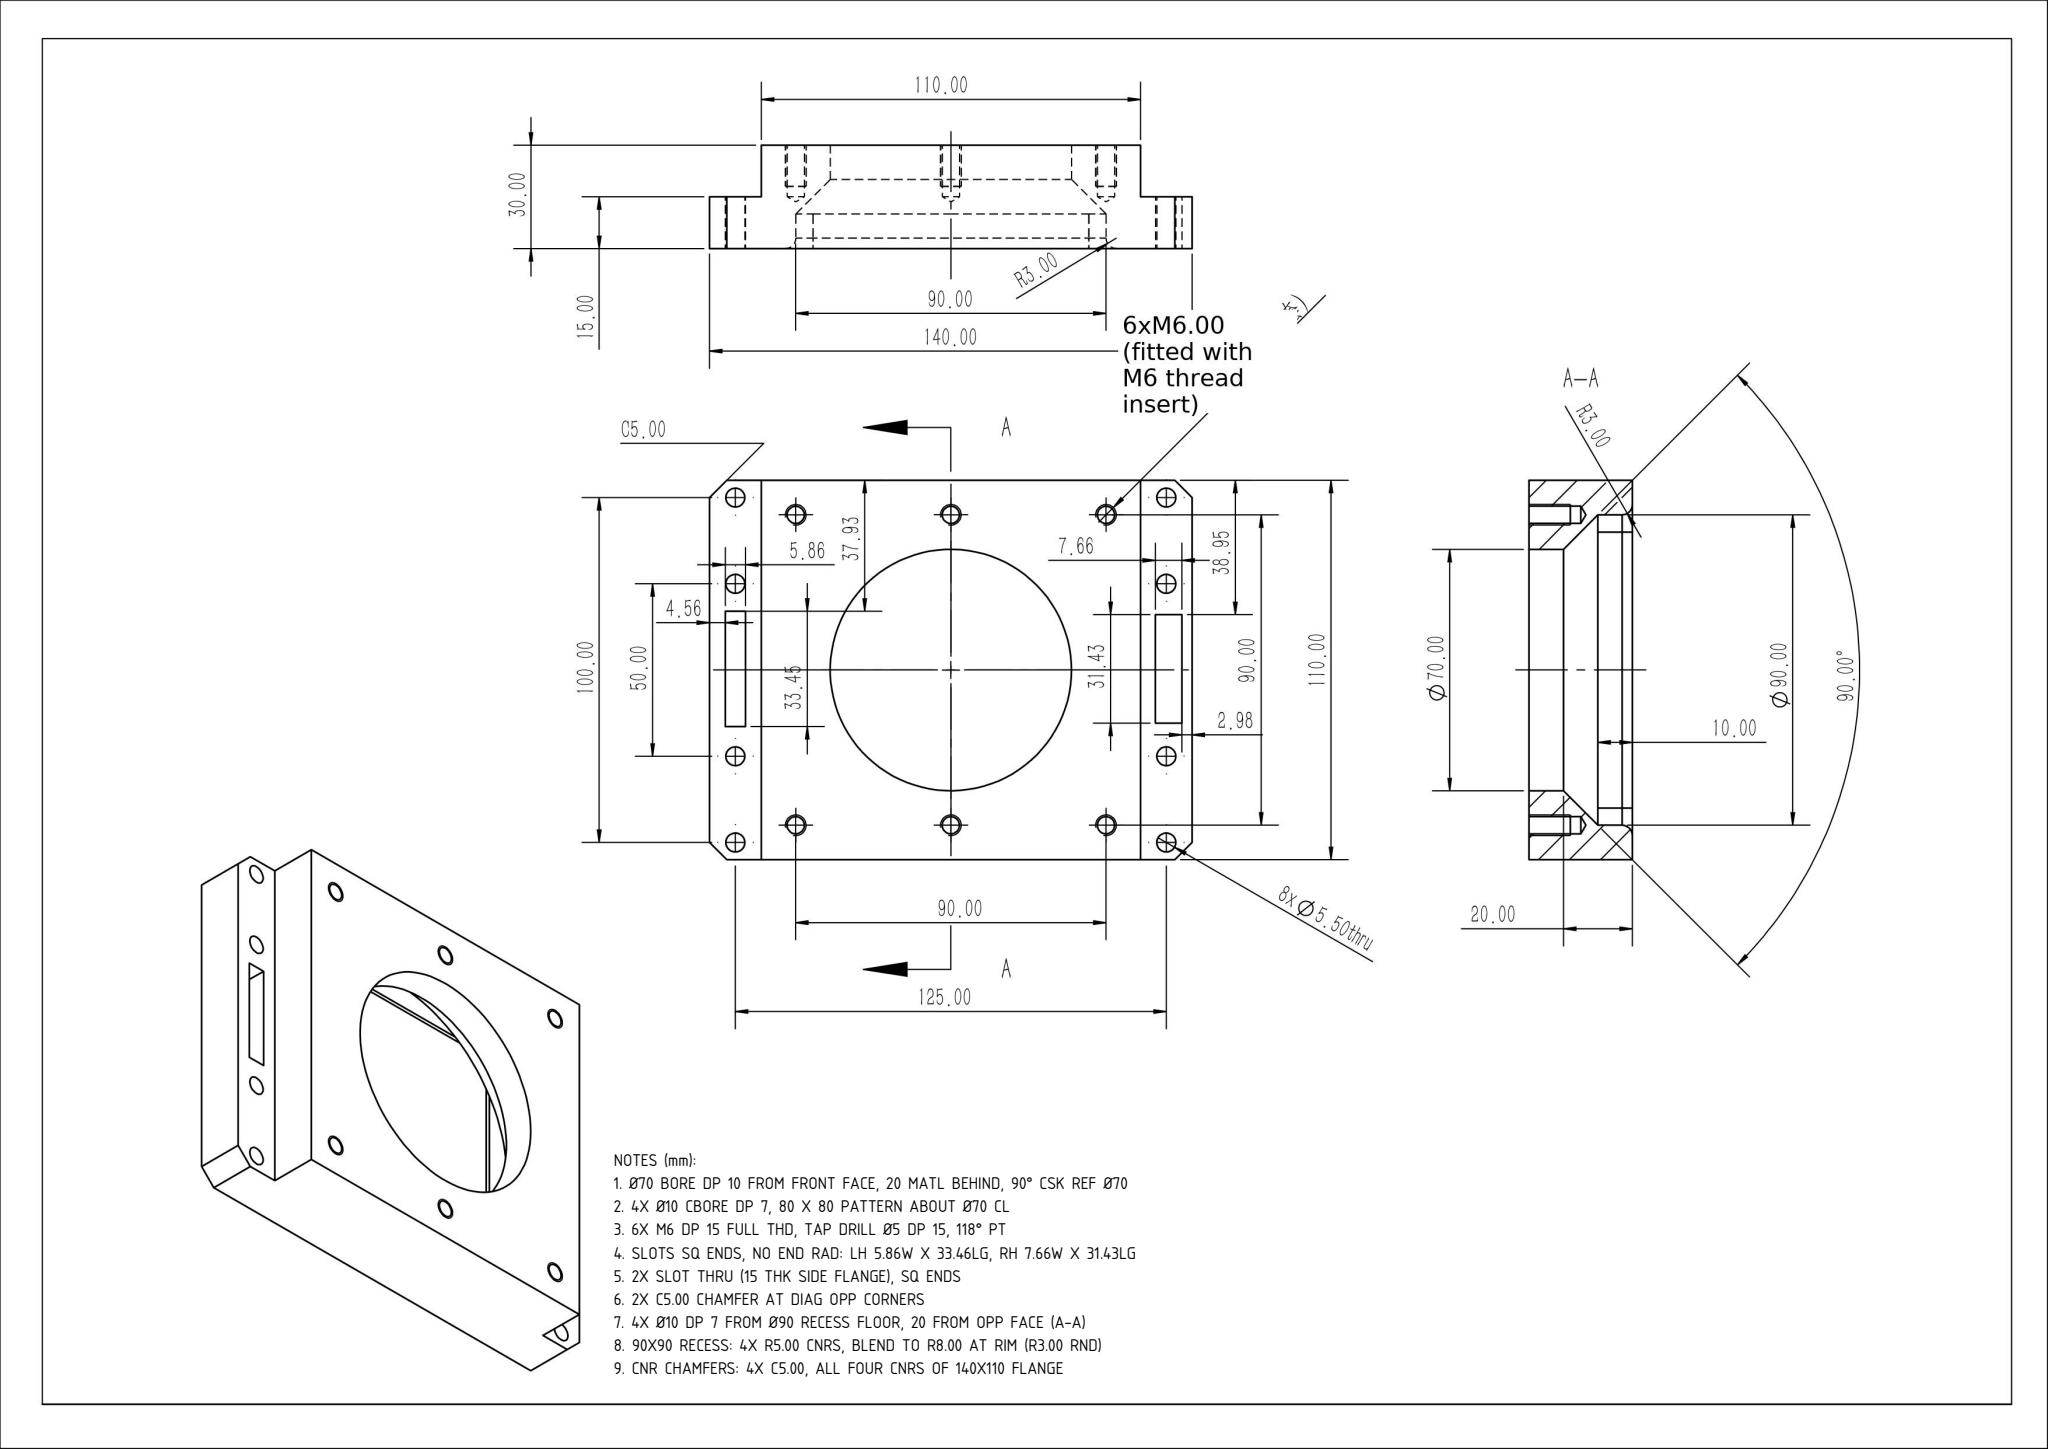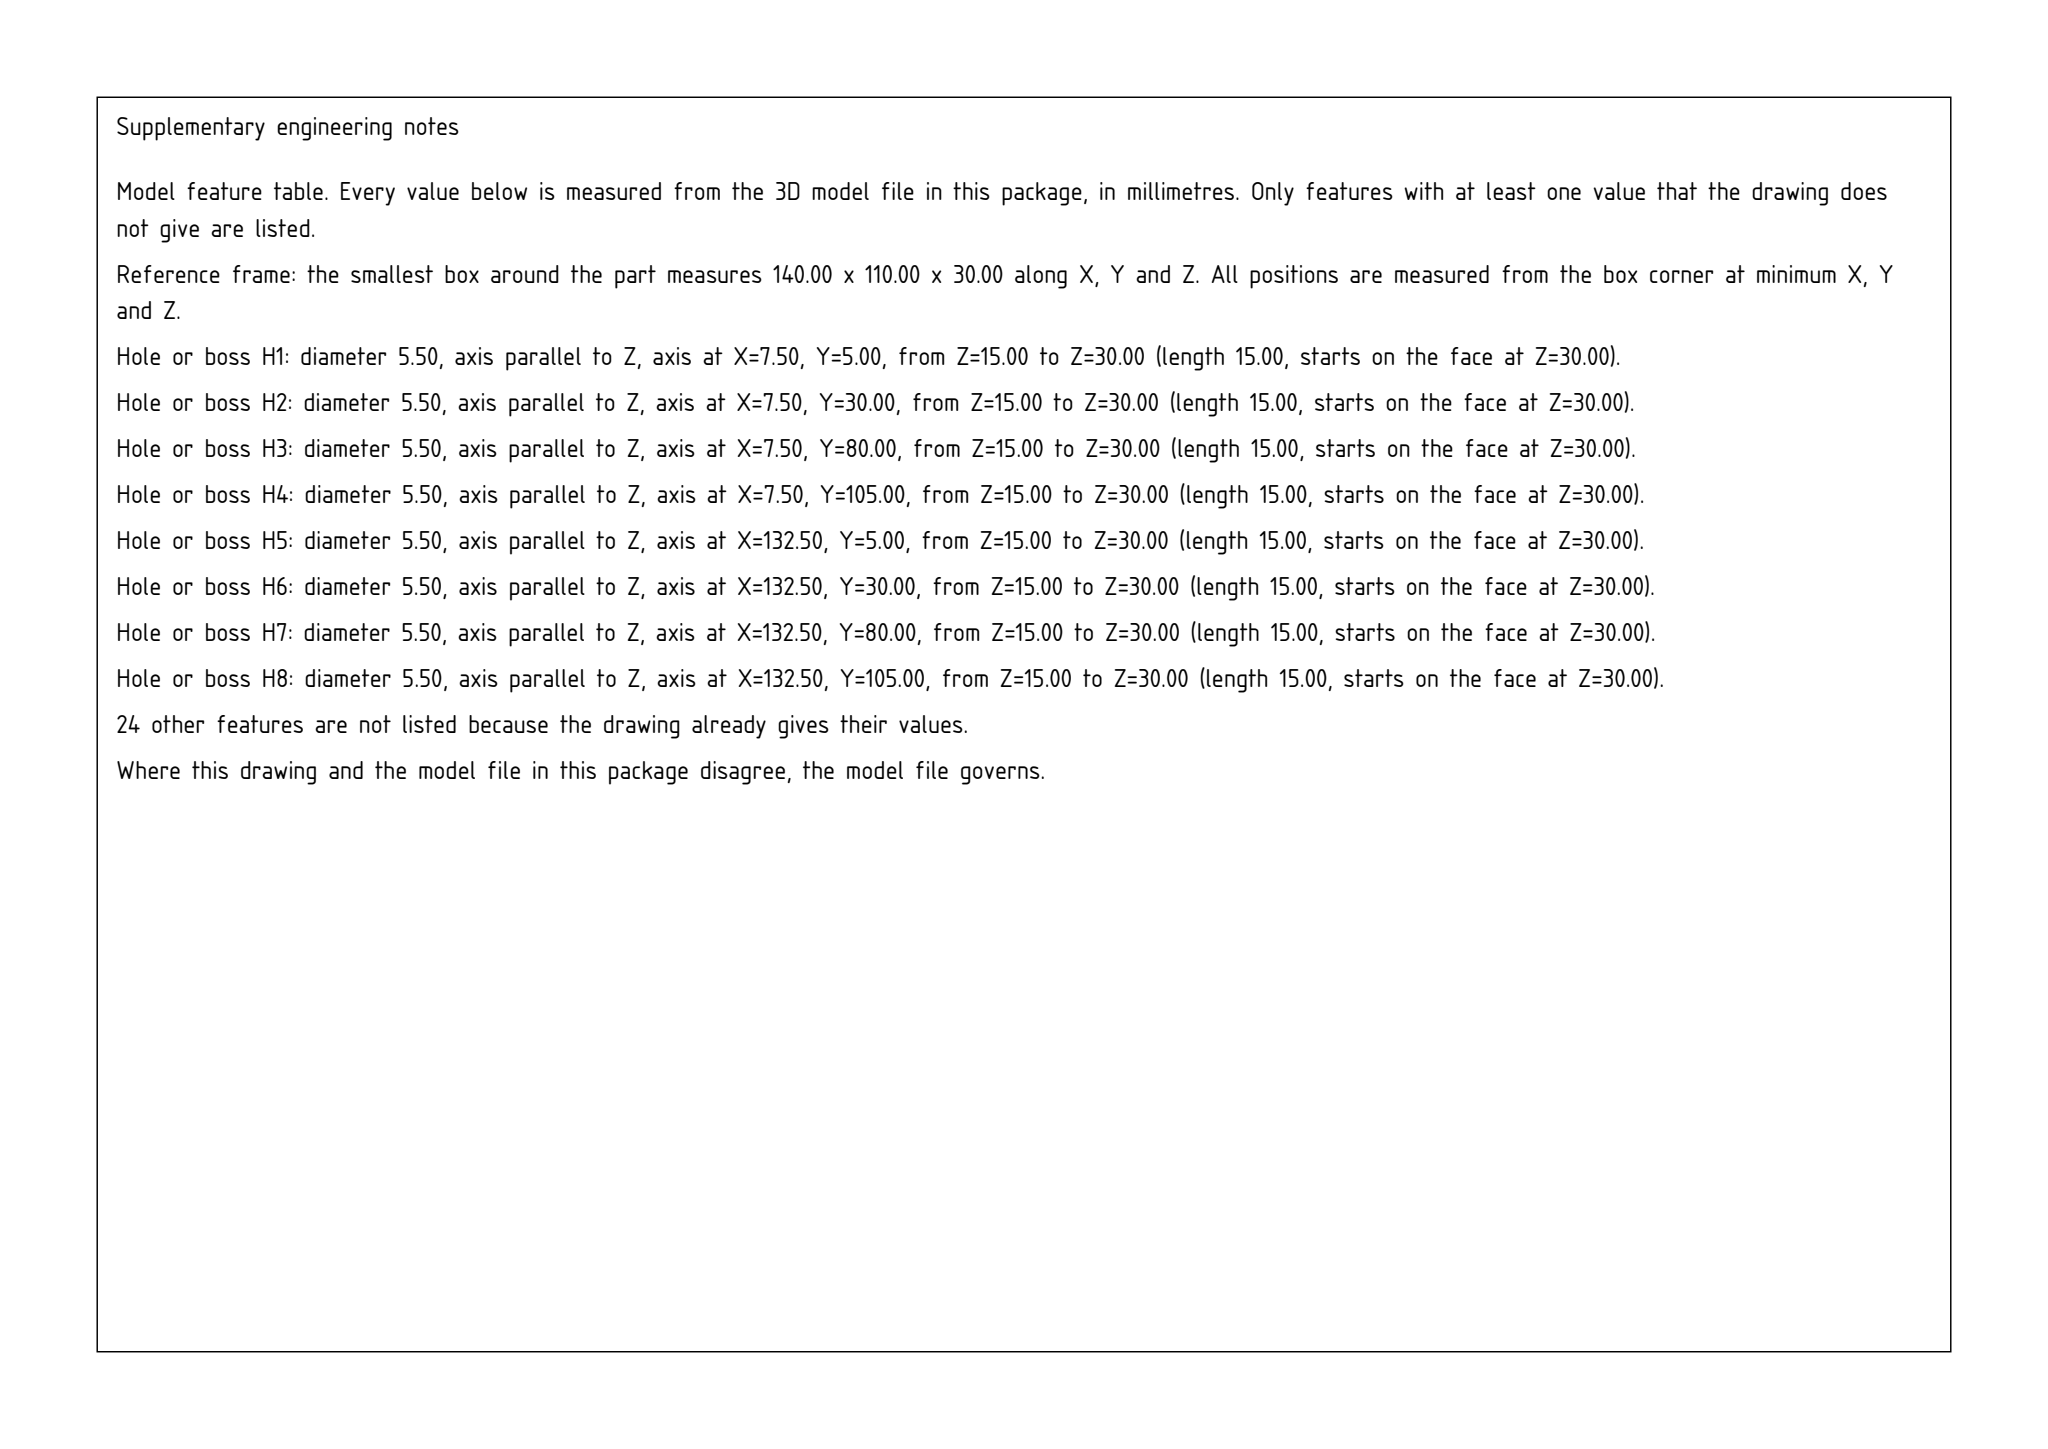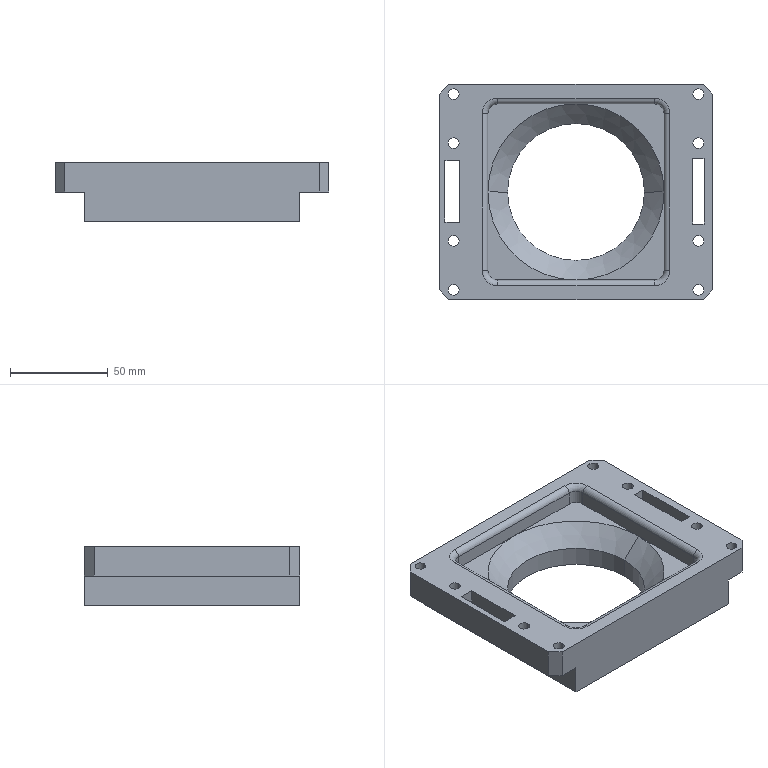Part | SolidWorks | mm | 1 solid | 86 faces | box 140 x 110 x 30 mm | volume 230039 mm3 | cylinder 38 | plane 30 | cone 14 | torus 4 | commonest cylinder face diameters 5.5 x16 5 x12 10 x4 6 x4 70 x2
Drawing notes:
Ø70 BORE DP 10 FROM FRONT FACE, 20 MATL BEHIND, 90° CSK REF Ø70 | from the solid: Cyl Ø70 axis z len 10 between z=20 and z=30 (bbox z=30); z planes 0/15/20/30; cone 90° ref Ø70
4X Ø10 CBORE DP 7, 80 X 80 PATTERN ABOUT Ø70 CL | from the solid: Cyl Ø10.0 axis z, len 7 at (30,15)(30,95)(110,15)(110,95); Ø70 axis at (70,55)
6X M6 DP 15 FULL THD, TAP DRILL Ø5 DP 15, 118° PT | from the solid: Cyl Ø5.0 axis z, len 15 at (25,10)(70,10)(115,10)(25,100)(70,100)(115,100); cones 118° ref Ø5 x12
SLOTS SQ ENDS, NO END RAD: LH 5.86W X 33.46LG, RH 7.66W X 31.43LG | from the solid: x planes 129.59/135.44 & 2.98/10.64; y planes 38.61/72.07 (33.46) & 39.62/71.05 (31.43); no slot-end fillets listed
2X SLOT THRU (15 THK SIDE FLANGE), SQ ENDS | from the solid: Slot walls only as x-planes 2.98/10.64 & 129.59/135.44 with y-planes 38.61/71.05 & 39.62/72.07; no z-plane floor between z=0 and z=15 flange faces, so slots break thru full 15 flange thickness
2X C5.00 CHAMFER AT DIAG OPP CORNERS | from the solid: Bbox 140 x 110 with corner cuts not appearing in axis_planes (oblique faces); two symmetric corner cuts present on 140x110 outline, size per existing C5.00 callout
4X Ø10 DP 7 FROM Ø90 RECESS FLOOR, 20 FROM OPP FACE (A-A) | from the solid: 4X Ø10 z-axis holes L=7 at (30,15),(110,15),(30,95),(110,95) = 80x80 about Ø70 CL (70,55); only candidate start face is the z=20 plane (4 corner faces of 90x90 recess at large end of 90deg cone to Ø70), 20 from z=0 face
90X90 RECESS: 4X R5.00 CNRS, BLEND TO R8.00 AT RIM (R3.00 RND) | from the solid: 4 concave arcs Ø10 (R5) z-axis at (30,15),(30,95),(110,15),(110,95) z20-27; tori minor_r 3.0 major 8.0 x4 at rim
CNR CHAMFERS: 4X C5.00, ALL FOUR CNRS OF 140X110 FLANGE | from the solid: 4 inclined planes 45/45 deg, size 5.0x5.0x15.0 at (0,0,15),(0,105,15),(135,0,15),(135,105,15)